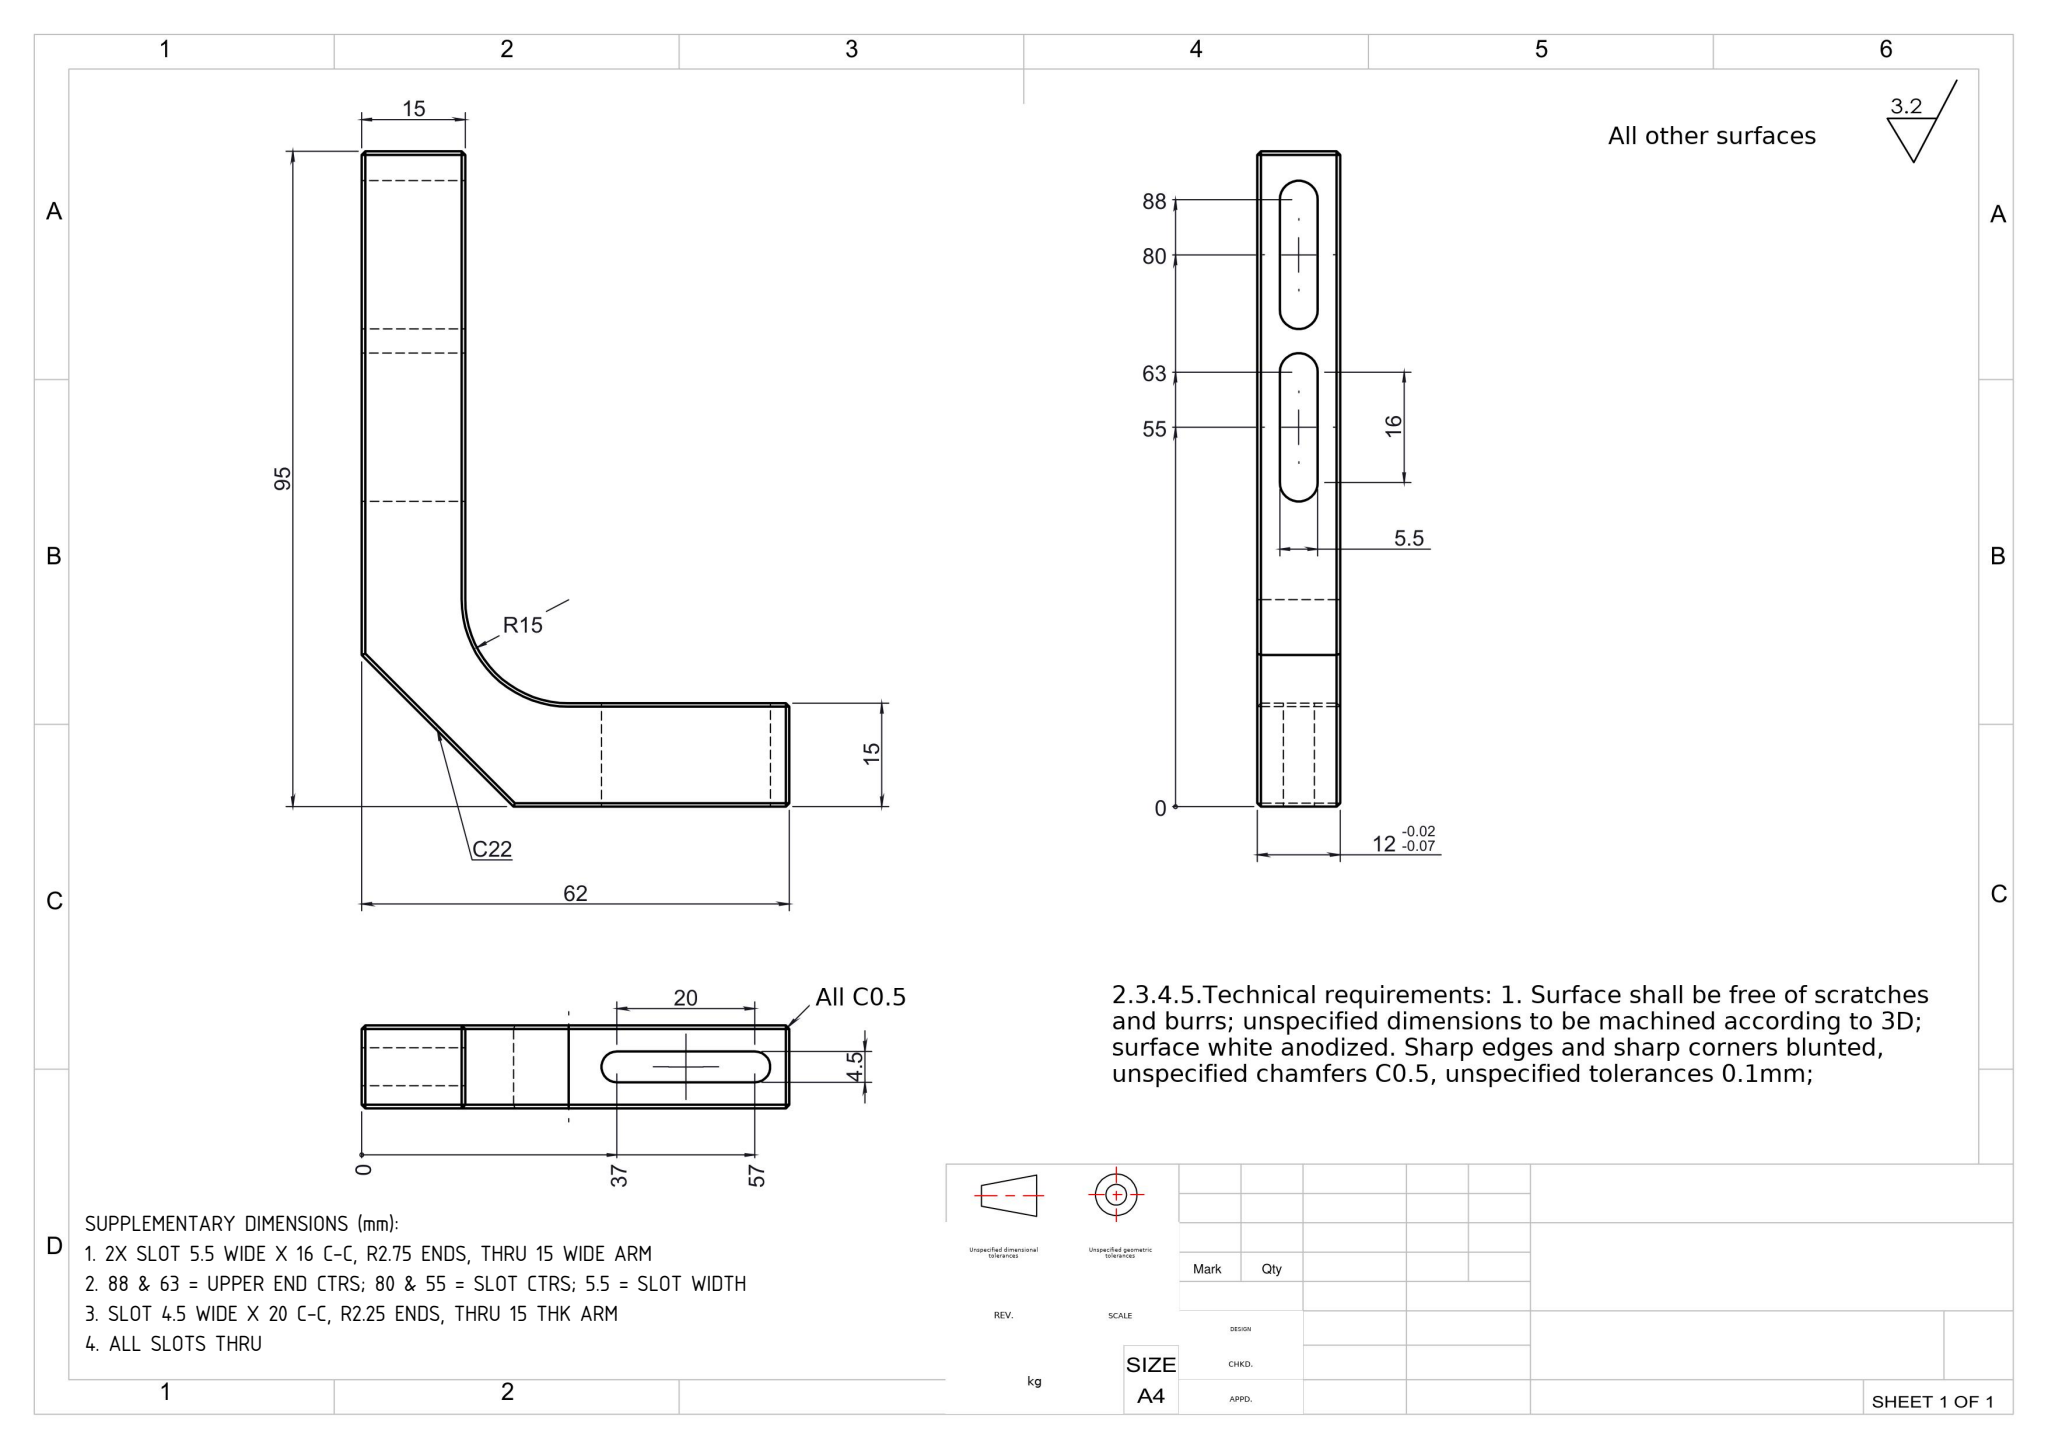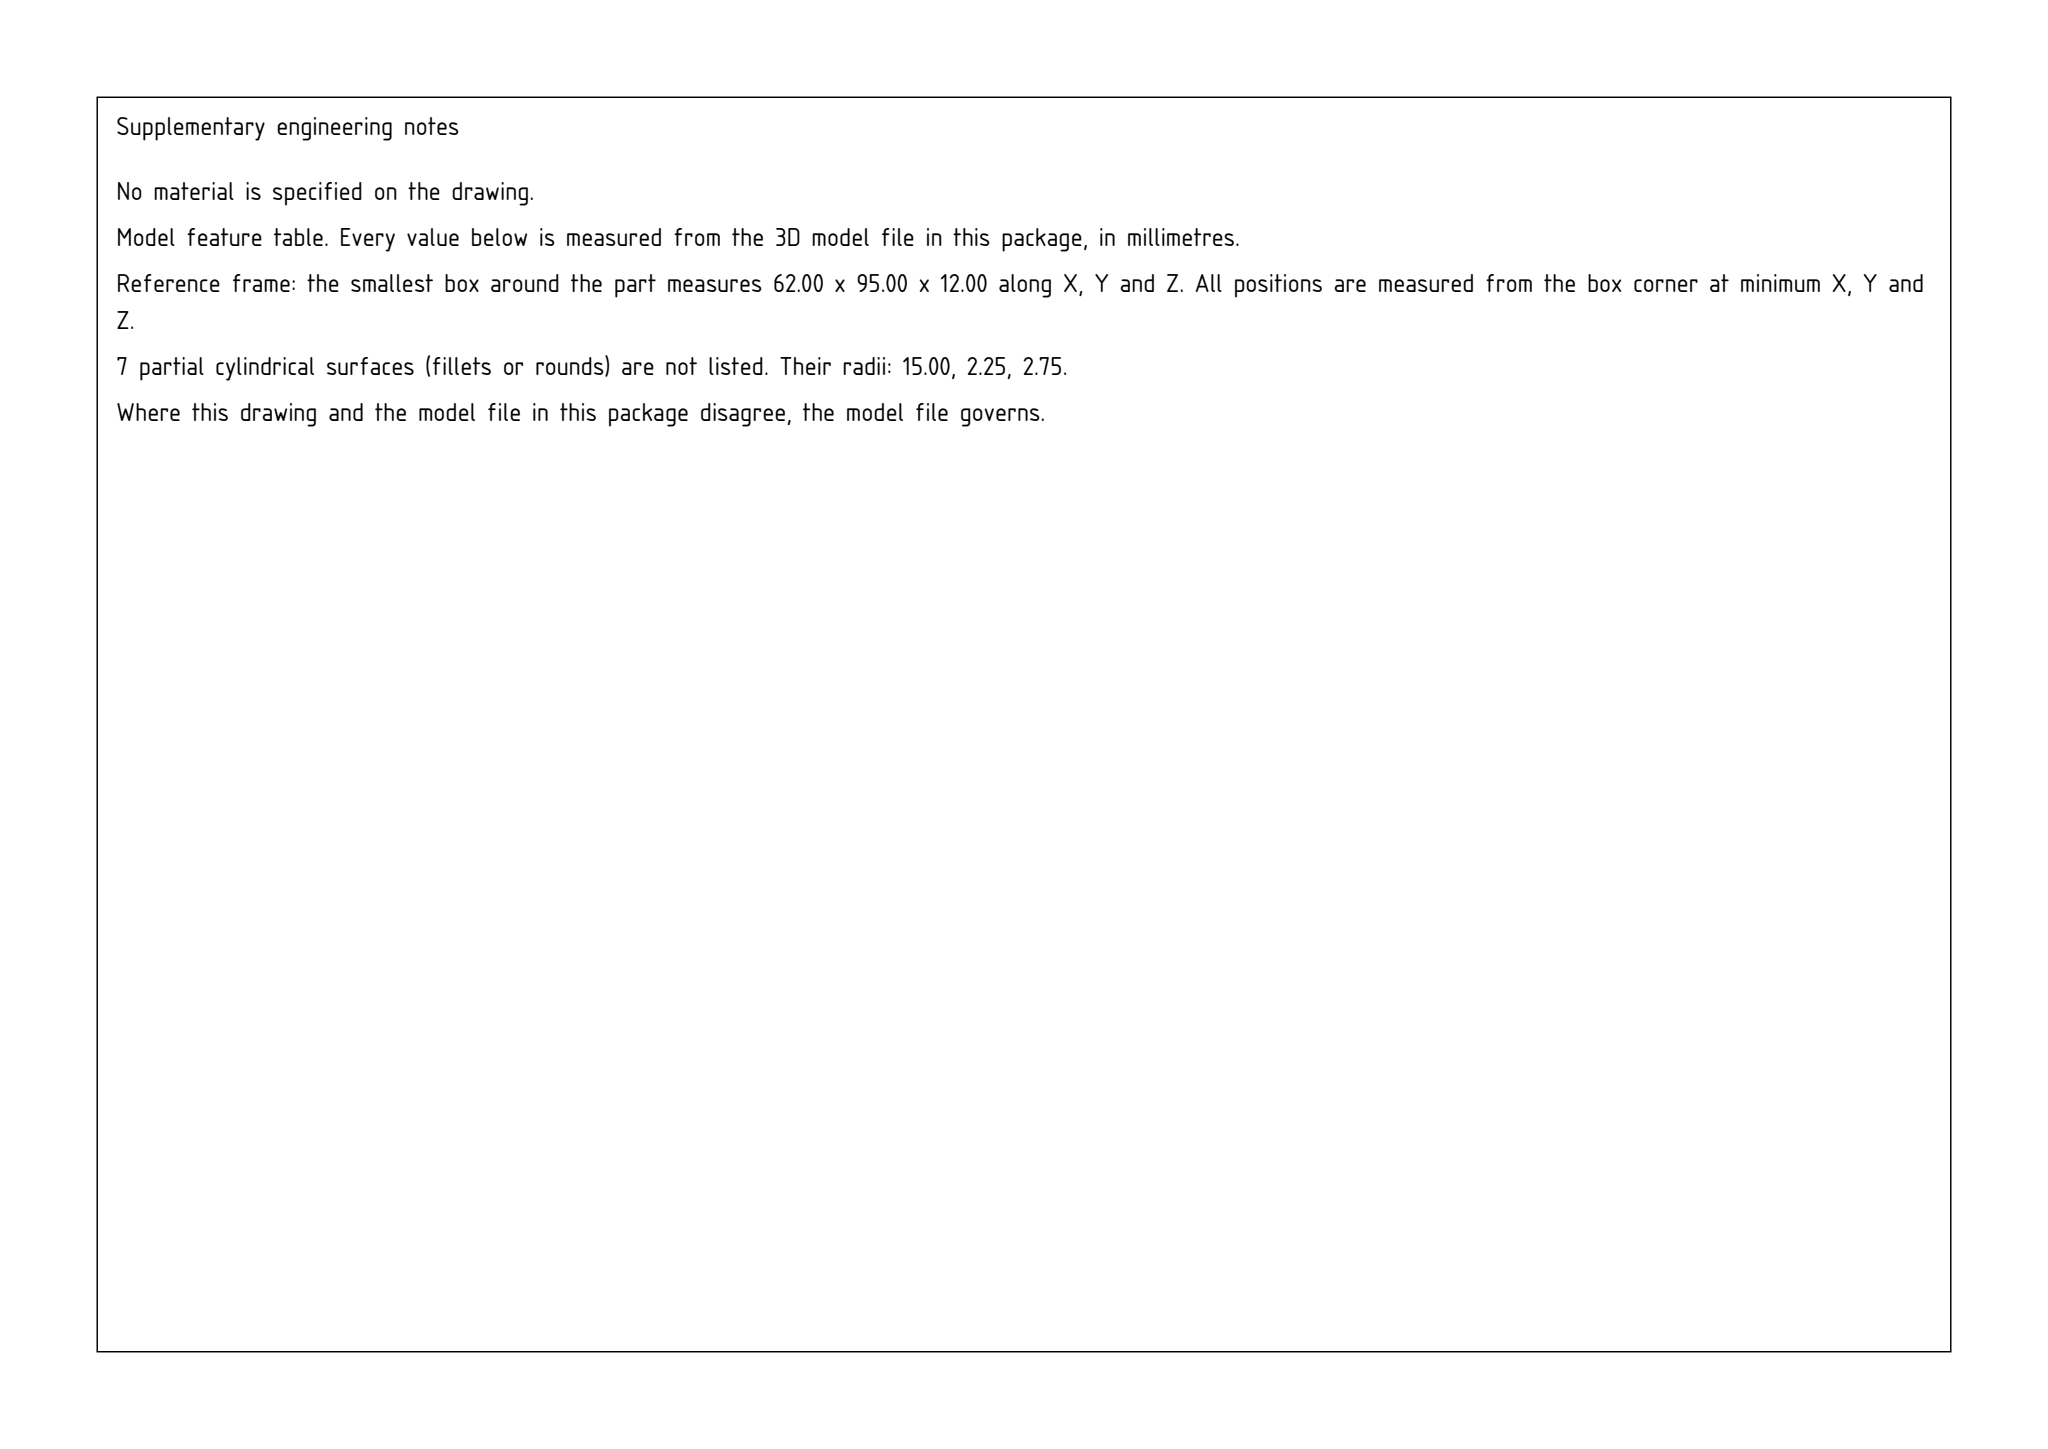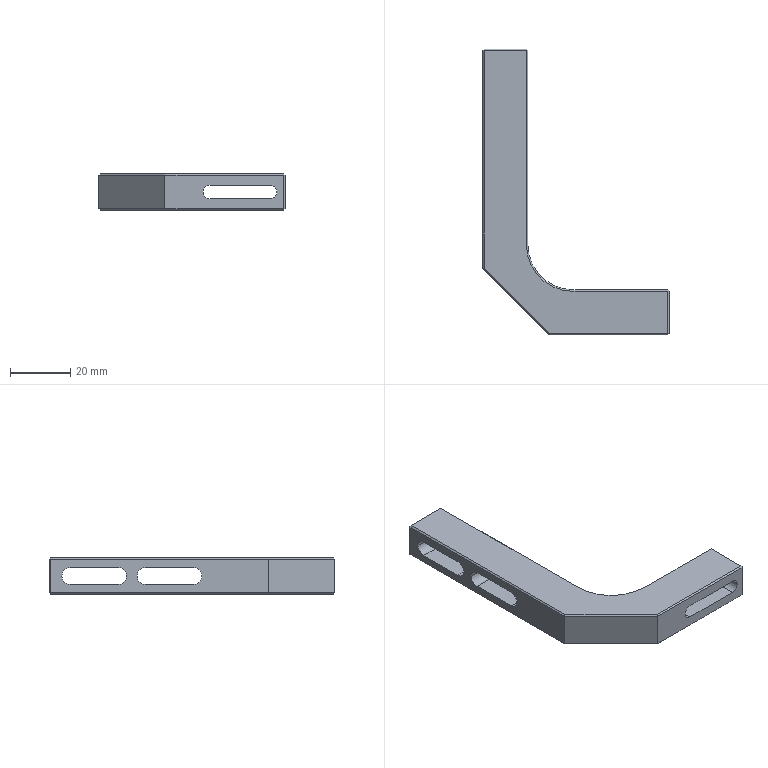Part | SolidWorks | mm | 1 solid | 53 faces | box 62 x 95 x 12 mm | volume 18215 mm3 | plane 41 | cylinder 10 | cone 2 | commonest cylinder face diameters 5.5 x6 4.5 x3 30 x1
build123d program:
from build123d import *

# Parameters (mm, degrees)
SKETCH1_W           = 62
SKETCH1_H           = 95
BOSS_EXTRUDE1_DEPTH = 12
SKETCH2_W           = 47
SKETCH2_H           = 80
CUT_EXTRUDE1_DEPTH  = 29
FILLET1_R           = 15
CUT_EXTRUDE2_DEPTH  = 29
CHAMFER1_SIZE       = 22
CHAMFER2_SIZE       = 0.5
CUT_EXTRUDE3_DEPTH  = 29


with BuildPart() as part:
    # Sketch1 → Boss-Extrude1 (new body)
    with BuildSketch(Plane.XY):
        Rectangle(SKETCH1_W, SKETCH1_H)
    extrude(amount=BOSS_EXTRUDE1_DEPTH)

    # Sketch2 → Cut-Extrude1 (cut)
    with BuildSketch(Plane.XY.offset(12)):
        with Locations((7.5, 7.5)):
            Rectangle(SKETCH2_W, SKETCH2_H)
    extrude(amount=-CUT_EXTRUDE1_DEPTH, mode=Mode.SUBTRACT)

    # Fillet1
    fillet1_edges = [part.edges().sort_by_distance(p)[0] for p in [
        (-16, -32.5, 6),
    ]]
    fillet(fillet1_edges, radius=FILLET1_R)

    # Sketch3 → Cut-Extrude2 (cut)
    with BuildSketch(Plane(origin=(0, -32.5, 0), x_dir=(1, 0, 0), z_dir=(0, 1, 0))):
        with BuildLine():
            Line((6, -3.75), (26, -3.75))
            ThreePointArc((26, -3.75), (28.25, -6), (26, -8.25))
            Line((26, -8.25), (6, -8.25))
            ThreePointArc((6, -8.25), (3.75, -6), (6, -3.75))
        make_face()
    extrude(amount=-CUT_EXTRUDE2_DEPTH, mode=Mode.SUBTRACT)

    # Chamfer1
    chamfer1_edges = [part.edges().sort_by_distance(p)[0] for p in [
        (-31, -47.5, 6),
    ]]
    chamfer(chamfer1_edges, length=CHAMFER1_SIZE)

    # Chamfer2
    chamfer2_edges = [part.edges().sort_by_distance(p)[0] for p in [
        (-31, 11, 12),
        (-23.5, 47.5, 0),
        (15, -32.5, 0),
        (-23.5, 47.5, 12),
        (31, -32.5, 6),
        (-16, 47.5, 6),
        (-16, 15, 12),
        (15, -32.5, 12),
        (-16, 15, 0),
        (-11.607, -28.107, 12),
        (-11.607, -28.107, 0),
        (31, -40, 12),
        (-31, 11, 0),
        (31, -40, 0),
        (11, -47.5, 0),
        (11, -47.5, 12),
        (-20, -36.5, 0),
        (-20, -36.5, 12),
        (31, -47.5, 6),
        (-31, 47.5, 6),
    ]]
    chamfer(chamfer2_edges, length=CHAMFER2_SIZE)

    # Sketch4 → Cut-Extrude3 (cut)
    with BuildSketch(Plane(origin=(-16, 0, 0), x_dir=(0, 0, -1), z_dir=(1, 0, 0))):
        with BuildLine():
            Line((-3.25, 40.5), (-3.25, 24.5))
            ThreePointArc((-3.25, 24.5), (-6, 21.75), (-8.75, 24.5))
            Line((-8.75, 24.5), (-8.75, 40.5))
            ThreePointArc((-8.75, 40.5), (-6, 43.25), (-3.25, 40.5))
        make_face()
        with BuildLine():
            Line((-3.25, 15.5), (-3.25, -0.5))
            ThreePointArc((-3.25, -0.5), (-6, -3.25), (-8.75, -0.5))
            Line((-8.75, -0.5), (-8.75, 15.5))
            ThreePointArc((-8.75, 15.5), (-6, 18.25), (-3.25, 15.5))
        make_face()
    extrude(amount=-CUT_EXTRUDE3_DEPTH, mode=Mode.SUBTRACT)


solid = part.part